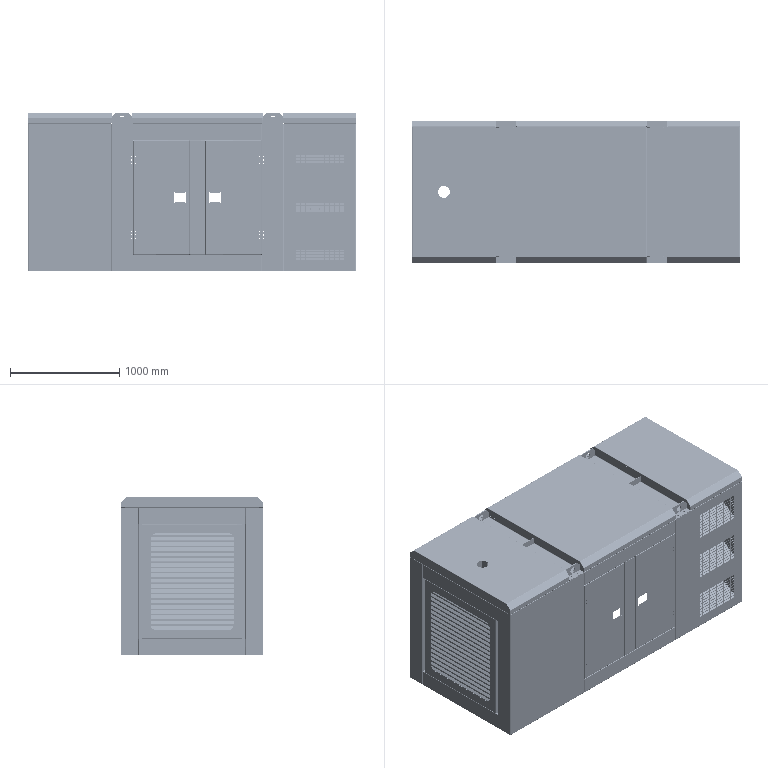Assembly | SolidWorks | mm | 126 component files | 130 solids | 11955 faces | box 3000 x 1300 x 1450 mm | volume 58582287 mm3 | plane 6546 | cylinder 5009 | spline 244 | cone 156 | commonest cylinder face diameters 6 x2539 10 x690 5 x576 8 x305 4 x293 9 x192 16 x116 7 x114
Bill of materials:
AirInletUpperBeam | 1 | Plain Carbon Steel | Rectangular panel with short bent flanges at the edges. A large grid of rectangular, rounded-corner slots sits in two equal side-by-side fields.
AirInletUpperBeamBaffle | 1 |  | Long prism-shaped shell with a vertical rear wall, two end walls and a sloped front face. The end profile is a right trapezoid.
AirInletVent | 1 | Plain Carbon Steel | Large rectangular panel with four fields of rectangular slots in a 2x2 layout. Narrow side flanges carry round holes.
AirInletVentBaffle | 2 |  | Long prism-shaped shell like unnamed part but with different proportions: rear wall, two end walls and a sloped front face.
Door | 4 | Plain Carbon Steel | Thin, flat rectangular plate with one rectangular cutout near one long edge and two groups of small oblong holes along the opposite long edge.
DoorStiffener | 8 | Plain Carbon Steel | Long straight channel with a C/U cross-section: a web and two parallel flanges with rounded bends.
BreakerDoor | 1 | Plain Carbon Steel | Thin, almost square flat plate. It has a central rounded-rectangle cutout, a rectangular cutout with slotted ends near one side, and four oblong slots along the opposite edge.
ElectricalCabinet | 1 | Plain Carbon Steel | Hat-section cover: a U-shaped box (face plus two side walls) with outward mounting flanges along both open edges. A horizontal obround slot runs through the face.
ElectricalCabinetBaffle | 1 | Plain Carbon Steel | Rectangular flat strip with a short bent lip at one end (L-profile). It has two round holes near the other end and one cylindrical boss or pin on the face.
CableClamp | 4 | Plain Carbon Steel | Thick U-shaped bracket or strap with a flat base, two parallel legs and radiused inner and outer bends.
ControlPanel | 1 | Plain Carbon Steel | Thin, flat rectangular plate with a large rectangular window, a narrow rectangular cutout with slotted ends, a row of three round holes, and four oblong slots along one edge.
ElectricalCabinetDoor | 1 | Plain Carbon Steel | Thin, flat rectangular plate with a large rounded-rectangle window near one end, a vertical obround slot, and four small slots along one long edge.
ElectricalCabinetDoorStiffener | 1 | Plain Carbon Steel | Long, straight C-channel profile of uniform thin wall. It has a flat web and two parallel flanges with rounded bends. No holes are visible.
ExhaustVent | 1 | Plain Carbon Steel | Square, thin frame-like plate with a large central opening shaped as a square with rounded corners. Narrow flanges or offset strips run along its edges, with small holes or slots spaced along two opposite edges.
Louver | 19 | Plain Carbon Steel | Long, narrow, thin strip bent along its length. In the end profile, a short straight leg joins a longer leg at an obtuse angle through a rounded bend.
FrontBeam | 2 | Plain Carbon Steel | Long, shallow, rectangular open tray or box section made of thin wall. A flat base has upturned walls on all four sides. Elongated slots are spaced along both long walls, and there are two slots in each end wall.
FrontSidePanel | 2 | Plain Carbon Steel | Large, flat, rectangular thin panel with a narrow return flange along one long edge and an L-shaped flange or lip along one end. Small holes run along the return flange, and slots are in the end flange.
FrontSidePanelReinforcementHorizontalRib | 2 |  | Long, straight L-angle profile of thin uniform wall. Two legs of about equal length meet at a rounded 90 degree bend. No holes are visible.
FrontSidePanelReinforcementVerticalRib | 2 |  | Long, slender L-angle profile with a rounded 90 degree bend. A single row of small holes runs along one leg.
hex nuts-style normal-grades ab gb | 12 |  | Hexagonal nut-like body with a central round through-bore. The hex corners are chamfered on both faces, which gives curved edges on the side faces.
FrontTopCover | 1 | Plain Carbon Steel | Large, rectangular thin cover plate with one round hole set off-center. A downturned flange with angled corner transitions runs along one edge, and a narrow flange with small holes and a return lip runs along an adjacent edge.
FrontTopCoverStiffener | 1 |  | Long, slender L-angle strip with a rounded 90 degree bend. Four elongated slots are evenly spaced along one leg.
HangingChannel | 2 | Plain Carbon Steel | Long U-channel or trough with a flat base, two tall parallel side walls and rounded bends. The ends of the side walls are cut at an angle. Small holes run along both side walls, and larger holes sit near each end of the base.
HangingChannelStiffener | 2 |  | Flat rectangular plate of uniform thickness. The two corners on one long edge are rounded, and the other two corners are square. No holes are visible.
LiftingLug | 4 | Plain Carbon Steel | Flat plate of constant thickness. Its outline has a straight bottom edge, two vertical sides and two angled (chamfered) upper corners. It has one large central round through-hole and a small rounded notch cut into the middle of the bottom edge.
HingeColumn | 4 | Plain Carbon Steel | Long, narrow formed sheet part. The end-on view shows a shallow U-shaped channel with a short outward-turned flange on one side. The base carries two obround slots at each end, and small hole groups appear along the side flange.
LiftingBasePlate | 8 | Plain Carbon Steel | Flat rectangular plate of uniform thickness with two obround through-slots, one near each end. Two corners are rounded and the opposite two are square.
LiftingVerticalBeam | 4 | Plain Carbon Steel | Long, straight, thin-walled U-channel with rounded inside and outside bends and a constant cross-section. No holes are visible.
LiftingVerticalBeamStiffener | 12 | Plain Carbon Steel | Plain flat rectangular plate of uniform thickness. Two corners on one long edge are rounded and there are no holes.
LongitudinalStiffeningChannelSteel | 2 | Plain Carbon Steel | Long, shallow, open-top tray or channel with low side walls and closed end walls. Each end wall has two obround slots.
MiddleBeam | 4 | Plain Carbon Steel | Long formed sheet beam. The end profile is a deep vertical web with a short return flange at the bottom and an offset upturned lip along the top. The top lip has a gap in the middle with two small slots, and the ends have bent tabs with two obround slots each.
MiddleColumn | 2 | Plain Carbon Steel | Long formed sheet profile shaped like a hat (top-hat). The section is a U-channel with outward flanges at both rims. The base has two obround slots at each end, and small holes are visible along one side.
MiddleTopCover | 1 | Plain Carbon Steel | Large, almost square flat panel with shallow formed edges on two opposite sides. The end view shows short angled bends that turn down into vertical lips, with a small return at one end. A row of small holes runs along one formed edge.
TopCoverStiffener | 2 | Plain Carbon Steel | Very long, slender C-shaped (lipless channel) profile with a rounded-corner rectangular section open on one side. No holes are visible.
RearLeftSidePlate | 1 | Plain Carbon Steel | L-shaped bent sheet panel. The large face has three rectangular grid arrays of small rectangular perforations, and the face meets a narrower side flange at a right-angle bend. Short edge returns and small holes or obround slots are present along the edges.
RearLeftSidePlateAirInletBaffle | 3 | Plain Carbon Steel | Thin sheet part with an open-box form: a back wall, two triangular or trapezoidal end walls, and a sloped base face. In the side view the profile tapers to a point. There are no holes or cutouts.
RearRightSidePanelVerticalRib1 | 1 | Plain Carbon Steel | Long, slender L-section angle strip that looks like bent sheet, with a rounded inside bend and three small holes evenly spaced along one leg.
RearRightSidePlate | 1 | Plain Carbon Steel | Flat rectangular panel that looks like bent sheet, with a large rectangular window cutout. It has one large round hole surrounded by four small holes near a top corner and a row of four round holes below the window. Its edges are folded into perimeter flanges, including a deeper flange down one long side, and the flanges carry small holes and oblong slots.
RearRightSidePlateDoorHorizontalRib | 2 | Plain Carbon Steel | Long narrow strip that looks like bent sheet: a flat top web with one long edge bent down into a flange. The web extends past the flange at both ends, forming end tabs or notches.
RearRightSidePlateDoorVerticalRib2 | 1 | Plain Carbon Steel | Long, slender L-section angle strip that looks like bent sheet, with a rounded inside bend and three small holes evenly spaced along one leg.
RearTopCover | 1 | Plain Carbon Steel | Shallow rectangular plate or cover with a flat top face and short side walls or flanges. The corners at both short ends are chamfered at an angle.
Mates:
1. coincident | FrontSidePlateAssembly-1/FrontSidePanel-1 face at (-416.713, -34.451, 675.478) dir (0, 0, -1) | FrontSidePlateAssembly-2/FrontSidePanel-1 face at (-416.713, 1223.549, 675.478) dir (0, 0, -1)
2. coincident | FrontSidePlateAssembly-1/FrontSidePanel-1 face at (-420.713, 123.549, 2025.478) dir (-1, 0, 0) | FrontSidePlateAssembly-2/FrontSidePanel-1 face at (-420.713, 1103.549, 675.478) dir (-1, 0, 0)
3. distance | FrontSidePlateAssembly-1/FrontSidePanel-1 face at (-420.713, -36.451, 2025.478) dir (0, -1, 0) | FrontSidePlateAssembly-2/FrontSidePanel-1 face at (-420.713, 1263.549, 675.478) dir (0, 1, 0)
4. coincident | FrontSidePlateAssembly-1/FrontSidePanel-1 face at (-420.713, -36.451, 2025.478) dir (0, -1, 0) | HingeColumn-1 face at (339.287, -36.451, 2025.478) dir (0, -1, 0)
5. coincident | FrontSidePlateAssembly-1/FrontSidePanel-1 face at (-416.713, -34.451, 675.478) dir (0, 0, -1) | HingeColumn-1 face at (343.287, -34.451, 675.478) dir (0, 0, -1)
6. coincident | FrontSidePlateAssembly-1/FrontSidePanel-1 face at (339.287, -36.451, 2025.478) dir (1, 0, 0) | HingeColumn-1 face at (339.287, 13.549, 2025.478) dir (-1, 0, 0)
7. coincident | HingeColumn-1 face at (343.287, -34.451, 675.478) dir (0, 0, -1) | MiddleBeam-1 face at (539.287, -36.451, 675.478) dir (0, 0, -1)
8. coincident | HingeColumn-1 face at (339.287, -36.451, 2025.478) dir (0, -1, 0) | MiddleBeam-1 face at (539.287, -36.451, 825.478) dir (0, -1, 0)
9. coincident | HingeColumn-1 face at (539.287, -36.451, 2025.478) dir (1, 0, 0) | MiddleBeam-1 face at (539.287, 3.549, 825.478) dir (-1, 0, 0)
10. coincident | MiddleBeam-1 face at (539.287, -36.451, 675.478) dir (0, 0, -1) | HingeColumn-2 face at (1915.287, 13.549, 675.478) dir (0, 0, -1)
11. coincident | MiddleBeam-1 face at (539.287, -36.451, 825.478) dir (0, -1, 0) | HingeColumn-2 face at (1919.287, -36.451, 675.478) dir (0, -1, 0)
12. coincident | MiddleBeam-1 face at (1719.287, 3.549, 825.478) dir (1, 0, 0) | HingeColumn-2 face at (1719.287, -36.451, 675.478) dir (-1, 0, 0)
13. coincident | HingeColumn-1 face at (539.287, -36.451, 2025.478) dir (1, 0, 0) | MiddleBeam-2 face at (539.287, 3.549, 1875.478) dir (-1, 0, 0)
14. coincident | HingeColumn-1 face at (339.287, -36.451, 2025.478) dir (0, -1, 0) | MiddleBeam-2 face at (1719.287, -36.451, 1875.478) dir (0, -1, 0)
15. coincident | HingeColumn-1 face at (343.287, 13.549, 2025.478) dir (0, 0, 1) | MiddleBeam-2 face at (1719.287, -36.451, 2025.478) dir (0, 0, 1)
16. coincident | MiddleBeam-1 face at (539.287, 3.549, 825.478) dir (0, 0, 1) | MiddleColumn-1 face at (1059.287, -34.451, 825.478) dir (0, 0, -1)
17. coincident | MiddleBeam-1 face at (539.287, -36.451, 825.478) dir (0, -1, 0) | MiddleColumn-1 face at (1059.287, -36.451, 1875.478) dir (0, -1, 0)
18. distance | HingeColumn-1 face at (539.287, -36.451, 2025.478) dir (1, 0, 0) | MiddleColumn-1 face at (1059.287, -34.451, 825.478) dir (-1, 0, 0)
19. coincident | HingeColumn-1 face at (339.287, -36.451, 2025.478) dir (0, -1, 0) | DoorAssembly-1/Door-1 face at (541.787, -36.451, 1872.978) dir (0, -1, 0)
20. distance | MiddleBeam-1 face at (539.287, 3.549, 825.478) dir (0, 0, 1) | DoorAssembly-1/Door-1 face at (541.787, -34.451, 827.978) dir (0, 0, -1)
21. distance | MiddleColumn-1 face at (1059.287, -34.451, 825.478) dir (-1, 0, 0) | DoorAssembly-1/Door-1 face at (1056.787, -34.451, 827.978) dir (1, 0, 0)
22. coincident | HingeColumn-2 face at (1919.287, -36.451, 675.478) dir (0, -1, 0) | DoorAssembly-2/Door-1 face at (1716.787, -36.451, 827.978) dir (0, -1, 0)
23. distance | HingeColumn-2 face at (1719.287, -36.451, 675.478) dir (-1, 0, 0) | DoorAssembly-2/Door-1 face at (1716.787, -34.451, 1872.978) dir (1, 0, 0)
24. distance | MiddleBeam-1 face at (539.287, 3.549, 825.478) dir (0, 0, 1) | DoorAssembly-2/Door-1 face at (1716.787, -34.451, 827.978) dir (0, 0, -1)
25. coincident | HingeColumn-2 face at (1915.287, 13.549, 677.478) dir (0, 0, 1) | LiftingVerticalBeamAssembly-1/LiftingBasePlate-2 face at (1753.287, -29.451, 677.478) dir (0, 0, -1)
26. coincident | HingeColumn-2 face at (1919.287, -34.451, 675.478) dir (0, 1, 0) | LiftingVerticalBeamAssembly-1/LiftingVerticalBeam-1 face at (1749.287, -34.451, 2022.478) dir (0, -1, 0)
27. distance | HingeColumn-2 face at (1919.287, 13.549, 675.478) dir (1, 0, 0) | LiftingVerticalBeamAssembly-1/LiftingVerticalBeam-1 face at (1889.287, -34.451, 2022.478) dir (1, 0, 0)
28. coincident | HingeColumn-1 face at (343.287, -34.451, 677.478) dir (0, 0, 1) | LiftingVerticalBeamAssembly-2/LiftingBasePlate-2 face at (373.287, -29.451, 677.478) dir (0, 0, -1)
29. coincident | HingeColumn-1 face at (339.287, -34.451, 2025.478) dir (0, 1, 0) | LiftingVerticalBeamAssembly-2/LiftingVerticalBeam-1 face at (369.287, -34.451, 2022.478) dir (0, -1, 0)
30. distance | HingeColumn-1 face at (339.287, 13.549, 2025.478) dir (-1, 0, 0) | LiftingVerticalBeamAssembly-2/LiftingVerticalBeam-1 face at (369.287, 19.549, 2022.478) dir (-1, 0, 0)
31. coincident | FrontSidePlateAssembly-1/FrontSidePanel-1 face at (-420.713, 123.549, 2025.478) dir (-1, 0, 0) | FrontBeam-1 face at (-420.713, 123.549, 675.478) dir (-1, 0, 0)
32. coincident | FrontSidePlateAssembly-1/FrontSidePanel-1 face at (-380.713, 123.549, 2025.478) dir (0, 1, 0) | FrontBeam-1 face at (-418.713, 123.549, 675.478) dir (0, -1, 0)
33. coincident | FrontSidePlateAssembly-2/FrontSidePanel-1 face at (-380.713, 1107.549, 675.478) dir (0, 0, -1) | FrontBeam-1 face at (-418.713, 123.549, 675.478) dir (0, 0, -1)
34. coincident | FrontSidePlateAssembly-1/FrontSidePanel-1 face at (-420.713, 123.549, 2025.478) dir (-1, 0, 0) | FrontBeam-2 face at (-420.713, 123.549, 1875.478) dir (-1, 0, 0)
35. coincident | FrontSidePlateAssembly-1/FrontSidePanel-1 face at (-380.713, 123.549, 2025.478) dir (0, 1, 0) | FrontBeam-2 face at (-418.713, 123.549, 1875.478) dir (0, -1, 0)
36. coincident | FrontSidePlateAssembly-1/FrontSidePanel-1 face at (-380.713, 119.549, 2025.478) dir (0, 0, 1) | FrontBeam-2 face at (-418.713, 123.549, 2025.478) dir (0, 0, 1)
37. coincident | FrontSidePlateAssembly-1/FrontSidePanel-1 face at (-420.713, 123.549, 2025.478) dir (-1, 0, 0) | ExhaustVentAssembly-1/ExhaustVent-1 face at (-420.713, 153.549, 1875.478) dir (-1, 0, 0)
38. coincident | FrontBeam-1 face at (-418.713, 123.549, 825.478) dir (0, 0, 1) | ExhaustVentAssembly-1/ExhaustVent-1 face at (-380.713, 153.549, 825.478) dir (0, 0, -1)
39. distance | FrontSidePlateAssembly-1/FrontSidePanel-1 face at (-380.713, 123.549, 2025.478) dir (0, 1, 0) | ExhaustVentAssembly-1/ExhaustVent-1 face at (-380.713, 153.549, 1875.478) dir (0, -1, 0)
40. coincident | MiddleColumn-3 face at (1199.287, 1263.549, 1875.478) dir (0, 1, 0) | DoorAssembly-4/Door-1 face at (541.787, 1263.549, 827.978) dir (0, 1, 0)
41. distance | HingeColumn-5 face at (539.287, 1263.549, 675.478) dir (1, 0, 0) | DoorAssembly-4/Door-1 face at (541.787, 1261.549, 1872.978) dir (-1, 0, 0)
42. distance | MiddleBeam-6 face at (1719.287, 1223.549, 825.478) dir (0, 0, 1) | DoorAssembly-4/Door-1 face at (541.787, 1261.549, 827.978) dir (0, 0, -1)
43. coincident | MiddleColumn-3 face at (1199.287, 1263.549, 1875.478) dir (0, 1, 0) | DoorAssembly-5/Door-1 face at (1716.787, 1263.549, 1872.978) dir (0, 1, 0)
44. distance | HingeColumn-6 face at (1719.287, 1263.549, 2025.478) dir (-1, 0, 0) | DoorAssembly-5/Door-1 face at (1716.787, 1261.549, 827.978) dir (1, 0, 0)
45. distance | MiddleBeam-5 face at (539.287, 1223.549, 1875.478) dir (0, 0, -1) | DoorAssembly-5/Door-1 face at (1716.787, 1261.549, 1872.978) dir (0, 0, 1)
46. coincident | HingeColumn-6 face at (1915.287, 1213.549, 2025.478) dir (0, 0, 1) | RearRightSidePlateAssembly-1/RearRightSidePlate-1 face at (1923.287, 1261.549, 2025.478) dir (0, 0, 1)
47. coincident | HingeColumn-6 face at (1919.287, 1263.549, 2025.478) dir (0, 1, 0) | RearRightSidePlateAssembly-1/RearRightSidePlate-1 face at (1919.287, 1263.549, 675.478) dir (0, 1, 0)
48. coincident | HingeColumn-6 face at (1919.287, 1213.549, 2025.478) dir (1, 0, 0) | RearRightSidePlateAssembly-1/RearRightSidePlate-1 face at (1919.287, 1263.549, 675.478) dir (-1, 0, 0)
49. coincident | HingeColumn-2 face at (1919.287, -36.451, 675.478) dir (0, -1, 0) | RearLeftSidePlateAssembly-2/RearLeftSidePlate-1 face at (1919.287, -36.451, 2025.478) dir (0, -1, 0)
50. coincident | HingeColumn-2 face at (1915.287, -34.451, 2025.478) dir (0, 0, 1) | RearLeftSidePlateAssembly-2/RearLeftSidePlate-1 face at (1923.287, 3.549, 2025.478) dir (0, 0, 1)
51. coincident | HingeColumn-2 face at (1919.287, 13.549, 675.478) dir (1, 0, 0) | RearLeftSidePlateAssembly-2/RearLeftSidePlate-1 face at (1919.287, -36.451, 2025.478) dir (-1, 0, 0)
52. coincident | RearLeftSidePlateAssembly-2/RearLeftSidePlate-1 face at (2539.287, -32.451, 2025.478) dir (0, 0, 1) | AirInletUpperBeamAssembly-1/AirInletUpperBeam-1 face at (2577.287, 1103.549, 2025.478) dir (0, 0, 1)
53. coincident | RearLeftSidePlateAssembly-2/RearLeftSidePlate-1 face at (2579.287, -36.451, 2025.478) dir (1, 0, 0) | AirInletUpperBeamAssembly-1/AirInletUpperBeam-1 face at (2579.287, 1103.549, 1625.478) dir (1, 0, 0)
54. coincident | RearRightSidePlateAssembly-1/RearRightSidePlate-1 face at (2579.287, 1103.549, 675.478) dir (0, -1, 0) | AirInletUpperBeamAssembly-1/AirInletUpperBeam-1 face at (2577.287, 1103.549, 1625.478) dir (0, 1, 0)
55. distance | RearRightSidePlateAssembly-1/RearRightSidePlate-1 face at (2539.287, 1259.549, 675.478) dir (0, 0, -1) | AirInletVentAssembly-1/AirInletVent-1 face at (2577.287, 154.549, 677.478) dir (0, 0, -1)
56. coincident | RearLeftSidePlateAssembly-2/RearLeftSidePlate-1 face at (2579.287, -36.451, 2025.478) dir (1, 0, 0) | AirInletVentAssembly-1/AirInletVent-1 face at (2579.287, 154.549, 677.478) dir (1, 0, 0)
57. distance | RearLeftSidePlateAssembly-2/RearLeftSidePlate-1 face at (2579.287, 123.549, 2025.478) dir (0, 1, 0) | AirInletVentAssembly-1/AirInletVent-1 face at (2544.287, 154.549, 677.478) dir (0, -1, 0)
58. coincident | RearRightSidePlateAssembly-1/RearRightSidePanelVerticalRib1-1 face at (1967.287, 1213.549, 677.978) dir (0, 1, 0) | ElectricalCabinetAssembly-1/CabinetAssembly-1/ElectricalCabinet-1 face at (2011.287, 1213.549, 1759.478) dir (0, -1, 0)
59. concentric | RearRightSidePlateAssembly-1/RearRightSidePlateDoorVerticalRib2-1 face at (2457.287, 1211.549, 1710.478) dir (0, 1, 0) r 5 | ElectricalCabinetAssembly-1/CabinetAssembly-1/ElectricalCabinet-1 face at (2457.287, 1205.549, 1710.478) dir (0, 1, 0) r 5
60. concentric | RearRightSidePlateAssembly-1/RearRightSidePanelVerticalRib1-1 face at (1981.287, 1211.549, 1710.478) dir (0, 1, 0) r 5 | ElectricalCabinetAssembly-1/CabinetAssembly-1/ElectricalCabinet-1 face at (1981.287, 1205.549, 1710.478) dir (0, 1, 0) r 5
61. coincident | RearRightSidePlateAssembly-1/RearRightSidePlate-1 face at (1919.287, 1263.549, 675.478) dir (0, 1, 0) | ElectricalCabinetDoorAssembly-1/ElectricalCabinetDoor-1 face at (1971.787, 1263.549, 927.978) dir (0, 1, 0)
62. distance | RearRightSidePlateAssembly-1/RearRightSidePlateDoorHorizontalRib-1 face at (1991.287, 1261.549, 1775.478) dir (0, 0, -1) | ElectricalCabinetDoorAssembly-1/ElectricalCabinetDoor-1 face at (1971.787, 1261.549, 1772.978) dir (0, 0, 1)
63. distance | RearRightSidePlateAssembly-1/RearRightSidePanelVerticalRib1-1 face at (1969.287, 1261.549, 677.978) dir (1, 0, 0) | ElectricalCabinetDoorAssembly-1/ElectricalCabinetDoor-1 face at (1971.787, 1261.549, 1772.978) dir (-1, 0, 0)
64. coincident | HingeColumn-5 face at (343.287, 1261.549, 2025.478) dir (0, 0, 1) | HangingChannelAssembly-2/HangingChannel-1 face at (539.287, 1263.549, 2025.478) dir (0, 0, -1)
65. coincident | HingeColumn-5 face at (339.287, 1263.549, 675.478) dir (0, 1, 0) | HangingChannelAssembly-2/HangingChannel-1 face at (539.287, 1263.549, 2029.478) dir (0, 1, 0)
66. coincident | HingeColumn-5 face at (339.287, 1213.549, 675.478) dir (-1, 0, 0) | HangingChannelAssembly-2/HangingChannel-1 face at (339.287, -36.451, 2029.478) dir (-1, 0, 0)
67. coincident | HingeColumn-6 face at (1915.287, 1213.549, 2025.478) dir (0, 0, 1) | HangingChannelAssembly-3/HangingChannel-1 face at (1719.287, -36.451, 2025.478) dir (0, 0, -1)
68. coincident | HingeColumn-6 face at (1919.287, 1263.549, 2025.478) dir (0, 1, 0) | HangingChannelAssembly-3/HangingChannel-1 face at (1719.287, 1263.549, 2029.478) dir (0, 1, 0)
69. coincident | HingeColumn-6 face at (1919.287, 1213.549, 2025.478) dir (1, 0, 0) | HangingChannelAssembly-3/HangingChannel-1 face at (1919.287, 1263.549, 2029.478) dir (1, 0, 0)
70. coincident | HangingChannelAssembly-3/HangingChannel-1 face at (1719.287, -36.451, 2025.478) dir (0, 0, -1) | LongitudinalStiffeningChannelSteel-1 face at (1719.287, 1191.549, 2025.478) dir (0, 0, -1)
71. coincident | HangingChannelAssembly-2/HangingChannel-1 face at (539.287, -36.451, 2122.478) dir (1, 0, 0) | LongitudinalStiffeningChannelSteel-1 face at (539.287, 1120.549, 2035.478) dir (-1, 0, 0)
72. distance | MiddleBeam-5 face at (539.287, 1263.549, 1875.478) dir (0, 1, 0) | LongitudinalStiffeningChannelSteel-1 face at (1719.287, 1191.549, 2025.478) dir (0, 1, 0)
73. coincident | FrontBeam-2 face at (-418.713, 123.549, 2025.478) dir (0, 0, 1) | FrontTopCoverAssembly-1/FrontTopCover-1 face at (339.287, 1263.549, 2025.478) dir (0, 0, -1)
74. coincident | FrontBeam-2 face at (-420.713, 123.549, 1875.478) dir (-1, 0, 0) | FrontTopCoverAssembly-1/FrontTopCover-1 face at (-420.713, 1211.892, 2123.478) dir (-1, 0, 0)
75. coincident | FrontSidePlateAssembly-1/FrontSidePanel-1 face at (-420.713, -36.451, 2025.478) dir (0, -1, 0) | FrontTopCoverAssembly-1/FrontTopCover-1 face at (-420.713, -36.451, 2025.478) dir (0, -1, 0)
76. coincident | MiddleBeam-2 face at (1719.287, -36.451, 2025.478) dir (0, 0, 1) | MiddleTopCoverAssembly-1/MiddleTopCover-1 face at (1719.287, 3.549, 2025.478) dir (0, 0, -1)
77. coincident | MiddleBeam-2 face at (1719.287, -36.451, 1875.478) dir (0, -1, 0) | MiddleTopCoverAssembly-1/MiddleTopCover-1 face at (1719.287, -36.451, 2025.478) dir (0, -1, 0)
78. distance | HangingChannelAssembly-3/HangingChannel-1 face at (1723.287, 1263.549, 2122.478) dir (1, 0, 0) | MiddleTopCoverAssembly-1/MiddleTopCover-1 face at (1724.287, 15.206, 2123.478) dir (-1, 0, 0)
79. coincident | RearLeftSidePlateAssembly-2/RearLeftSidePlate-1 face at (1923.287, 3.549, 2025.478) dir (0, 0, 1) | RearTopCoverAssembly-1/RearTopCover-1 face at (2579.287, 3.549, 2025.478) dir (0, 0, -1)
80. coincident | AirInletUpperBeamAssembly-1/AirInletUpperBeam-1 face at (2579.287, 1103.549, 1625.478) dir (1, 0, 0) | RearTopCoverAssembly-1/RearTopCover-1 face at (2579.287, 15.206, 2123.478) dir (1, 0, 0)
81. coincident | RearLeftSidePlateAssembly-2/RearLeftSidePlate-1 face at (1919.287, -36.451, 2025.478) dir (0, -1, 0) | RearTopCoverAssembly-1/RearTopCover-1 face at (2579.287, -36.451, 2025.478) dir (0, -1, 0)
82. coincident | AirInletUpperBeam-1 face at (-738.997, 97.614, 1368.825) dir (0, 1, 0) | AirInletUpperBeamBaffle-2 face at (185.003, 97.614, 1023.825) dir (0, -1, 0)
83. distance | AirInletUpperBeam-1 face at (-656.997, 97.614, 1272.325) dir (1, 0, 0) | AirInletUpperBeamBaffle-2 face at (-682.997, 247.614, 1227.222) dir (1, 0, 0)
84. distance | AirInletUpperBeam-1 face at (-384.497, 97.614, 1078.825) dir (0, 0, 1) | AirInletUpperBeamBaffle-2 face at (185.003, 249.614, 1023.825) dir (0, 0, -1)
85. coincident | AirInletVent-1 face at (-651.143, 76.053, 1533) dir (0, 1, 0) | AirInletVentBaffle-4 face at (-537.707, 76.053, 640) dir (0, -1, 0)
86. distance | AirInletVentBaffle-4 face at (-538.861, 196.053, 640) dir (0, 0, -1) | AirInletVent-1 face at (74.857, 76.053, 666) dir (0, 0, 1)
87. distance | AirInletVent-1 face at (-318.143, 76.053, 939) dir (-1, 0, 0) | AirInletVentBaffle-4 face at (-268.143, 198.053, 1510) dir (1, 0, 0)
88. parallel | Door-1 face at (207.586, 100.107, 573.135) dir (1, 0, 0) | DoorStiffener-1 face at (-297.414, 118.107, 1294.135) dir (-1, 0, 0)
89. distance | DoorStiffener-1 face at (-297.414, 118.107, 1294.135) dir (-1, 0, 0) | Door-1 face at (-307.414, 100.107, 573.135) dir (-1, 0, 0)
90. coincident | Door-1 face at (-307.414, 100.107, 1618.135) dir (0, 1, 0) | DoorStiffener-1 face at (-297.414, 100.107, 1298.135) dir (0, -1, 0)
91. distance | DoorStiffener-1 face at (-297.414, 120.107, 1298.135) dir (0, 0, 1) | Door-1 face at (-307.414, 100.107, 1618.135) dir (0, 0, 1)
92. coincident | Door-1 face at (-307.414, 100.107, 1618.135) dir (0, 1, 0) | DoorStiffener-2 face at (-302.414, 100.107, 933.135) dir (0, -1, 0)
93. distance | DoorStiffener-2 edge at (197.586, 116.107, 933.135) dir (0, -1, 0) | Door-1 face at (207.586, 100.107, 573.135) dir (1, 0, 0)
94. distance | Door-1 face at (-307.414, 100.107, 573.135) dir (0, 0, -1) | DoorStiffener-2 face at (-302.414, 100.107, 893.135) dir (0, 0, -1)
95. coincident | CabinetAssembly-1/ElectricalCabinet-1 face at (-270.686, -48.594, 510) dir (0, -1, 0) | ControlPanelAssembly-1/ControlPanel-1 face at (-268.186, -48.594, 1328) dir (0, 1, 0)
96. coincident | CabinetAssembly-1/ElectricalCabinet-1 face at (-270.686, -60.594, 1328) dir (0, 0, 1) | ControlPanelAssembly-1/ControlPanel-1 face at (143.814, -60.594, 1328) dir (0, 0, 1)
97. distance | CabinetAssembly-1/ElectricalCabinet-1 face at (-270.686, -60.594, 1328) dir (1, 0, 0) | ControlPanelAssembly-1/ControlPanel-1 face at (-268.186, -60.594, 1328) dir (-1, 0, 0)
98. coincident | CabinetAssembly-1/ElectricalCabinetBaffle-1 face at (-269.686, -48.594, 971) dir (0, -1, 0) | BreakerDoor-2 face at (143.814, -48.594, 512.5) dir (0, 1, 0)
99. distance | BreakerDoor-2 face at (143.814, -60.594, 965.5) dir (0, 0, 1) | ControlPanelAssembly-1/ControlPanel-1 face at (143.814, -60.594, 968) dir (0, 0, -1)
100. distance | CabinetAssembly-1/ElectricalCabinet-1 face at (-270.686, -60.594, 1328) dir (1, 0, 0) | BreakerDoor-2 face at (-268.186, -60.594, 965.5) dir (-1, 0, 0)
101. coincident | ElectricalCabinet-1 face at (-321.77, 87.808, 1338) dir (0, -1, 0) | ElectricalCabinetBaffle-1 face at (-318.77, 87.808, 983) dir (0, 1, 0)
102. coincident | ElectricalCabinet-1 face at (94.23, 87.808, 1338) dir (-1, 0, 0) | ElectricalCabinetBaffle-1 face at (94.23, 85.808, 983) dir (1, 0, 0)
103. distance | ElectricalCabinetBaffle-1 face at (-318.77, 85.808, 983) dir (0, 0, 1) | ElectricalCabinet-1 face at (-321.77, -52.192, 1338) dir (0, 0, 1)
104. coincident | ControlPanel-1 face at (-322.995, -149.043, 466.32) dir (0, 0, -1) | CableClamp-1 face at (-129.995, -109.043, 466.32) dir (0, 0, 1)
105. distance | ControlPanel-1 face at (-23.995, -79.043, 466.32) dir (0, 1, 0) | CableClamp-1 face at (-105.995, -109.043, 460.32) dir (0, 1, 0)
106. distance | CableClamp-1 face at (-131.995, -109.043, 466.32) dir (-1, 0, 0) | ControlPanel-1 face at (-322.995, -149.043, 468.32) dir (-1, 0, 0)
107. coincident | ControlPanel-1 face at (-322.995, -149.043, 466.32) dir (0, 0, -1) | CableClamp-2 face at (-244.995, -22.043, 466.32) dir (0, 0, 1)
108. distance | CableClamp-2 face at (-244.995, 1.957, 460.32) dir (-1, 0, 0) | ControlPanel-1 face at (-209.995, -79.043, 466.32) dir (1, 0, 0)
109. distance | ControlPanel-1 face at (-23.995, -79.043, 466.32) dir (0, 1, 0) | CableClamp-2 face at (-244.995, -24.043, 466.32) dir (0, -1, 0)
110. coincident | ElectricalCabinetDoor-1 face at (-422.942, 43.551, 1368.135) dir (0, 1, 0) | ElectricalCabinetDoorStiffener-1 face at (67.058, 43.551, 921.135) dir (0, -1, 0)
111. distance | ElectricalCabinetDoorStiffener-1 face at (-412.942, 61.551, 919.135) dir (-1, 0, 0) | ElectricalCabinetDoor-1 face at (-422.942, 43.551, 523.135) dir (-1, 0, 0)
112. distance | ElectricalCabinetDoor-1 face at (-422.942, 43.551, 523.135) dir (0, 0, -1) | ElectricalCabinetDoorStiffener-1 face at (67.058, 63.551, 883.135) dir (0, 0, -1)
113. coincident | ExhaustVent-1 face at (-628.17, 92.803, 1536) dir (0, 1, 0) | Louver-1 face at (351.83, 92.803, 1533) dir (0, -1, 0)
114. distance | Louver-1 face at (351.83, 94.803, 1533) dir (1, 0, 0) | ExhaustVent-1 face at (421.83, 130.803, 1536) dir (1, 0, 0)
115. distance | Louver-1 face at (338.487, 96.803, 619) dir (0, 0, -1) | ExhaustVent-1 face at (421.83, 92.803, 618) dir (0, 0, 1)
116. coincident | FrontSidePanel-1 face at (-740.849, 8.457, 2125.478) dir (0, 1, 0) | FrontSidePanelReinforcementVerticalRib-1 face at (-538.849, 8.457, 2122.978) dir (0, -1, 0)
117. distance | FrontSidePanel-1 face at (-740.849, 166.457, 2125.478) dir (-1, 0, 0) | FrontSidePanelReinforcementVerticalRib-1 face at (-540.849, 48.457, 2122.978) dir (-1, 0, 0)
118. distance | FrontSidePanelReinforcementVerticalRib-1 face at (-542.849, 12.457, 2122.978) dir (0, 0, 1) | FrontSidePanel-1 face at (-736.849, 46.457, 2123.478) dir (0, 0, -1)
119. coincident | FrontSidePanel-1 face at (-740.849, 8.457, 2125.478) dir (0, 1, 0) | FrontSidePanelReinforcementHorizontalRib-1 face at (-538.849, 8.457, 1425.478) dir (0, -1, 0)
120. coincident | FrontSidePanelReinforcementVerticalRib-1 face at (-538.849, 48.457, 2122.978) dir (1, 0, 0) | FrontSidePanelReinforcementHorizontalRib-1 face at (-538.849, 12.457, 1423.478) dir (-1, 0, 0)
121. distance | FrontSidePanelReinforcementHorizontalRib-1 face at (-538.849, 8.457, 1425.478) dir (0, 0, 1) | FrontSidePanel-1 face at (-736.849, 46.457, 2125.478) dir (0, 0, 1)
122. coincident | FrontSidePanel-1 face at (-698.849, 194.457, 2125.478) dir (1, 0, 0) | hex nuts-style normal-grades ab gb-1 face at (-698.849, 153.957, 959.601) dir (-1, 0, 0)
123. concentric | FrontSidePanel-1 face at (-698.849, 181.457, 975.478) dir (-1, 0, 0) r 4.5 | hex nuts-style normal-grades ab gb-1 face at (-698.849, 181.457, 975.478) dir (1, 0, 0) r 17.5
124. coincident | FrontTopCover-1 face at (-723.209, 181.253, 1683.5) dir (0, -1, 0) | FrontTopCoverStiffener-1 face at (-723.209, 181.253, 1483.5) dir (0, 1, 0)
125. distance | FrontTopCover-1 face at (-721.552, 181.253, 1683.5) dir (0, 0, 1) | FrontTopCoverStiffener-1 face at (-723.209, 181.253, 1483.5) dir (0, 0, 1)
126. distance | FrontTopCover-1 face at (-773.209, 83.253, 1683.5) dir (-1, 0, 0) | FrontTopCoverStiffener-1 face at (-723.209, 179.253, 1479.5) dir (-1, 0, 0)
127. coincident | HangingChannel-1 face at (-338.973, 553, 1544.5) dir (0, 0, -1) | LiftingLug-2 face at (-334.973, -683, 1544.5) dir (0, 0, 1)
128. coincident | HangingChannel-1 face at (-142.973, -747, 1544.5) dir (-1, 0, 0) | LiftingLug-2 face at (-142.973, -683, 1544.5) dir (1, 0, 0)
129. distance | LiftingLug-2 face at (-334.973, -693, 1544.5) dir (0, -1, 0) | HangingChannel-1 face at (-142.973, -743, 1544.5) dir (0, -1, 0)
130. coincident | HangingChannel-1 face at (-338.973, 553, 1544.5) dir (0, 0, -1) | HangingChannelStiffener-1 face at (-324.973, -94.5, 1544.5) dir (0, 0, 1)
131. coincident | HangingChannel-1 face at (-334.973, -747, 1451.5) dir (1, 0, 0) | HangingChannelStiffener-1 face at (-334.973, -94.5, 1534.5) dir (-1, 0, 0)
132. distance | HangingChannelStiffener-1 face at (-324.973, -99.5, 1534.5) dir (0, -1, 0) | HangingChannel-1 face at (-338.973, -747, 1544.5) dir (0, -1, 0)
133. coincident | LiftingVerticalBeam-1 face at (-75.046, -16.757, 745) dir (0, 0, 1) | LiftingBasePlate-1 face at (-80.046, -15.757, 745) dir (0, 0, 1)
134. coincident | LiftingVerticalBeam-1 face at (51.954, 33.243, 745) dir (0, 1, 0) | LiftingBasePlate-1 face at (-80.046, 33.243, 740) dir (0, 1, 0)
135. coincident | LiftingVerticalBeam-1 face at (51.954, -20.757, 745) dir (-1, 0, 0) | LiftingBasePlate-1 face at (51.954, 33.243, 740) dir (1, 0, 0)
136. coincident | LiftingVerticalBeam-1 face at (46.954, -16.757, -600) dir (0, 0, -1) | LiftingBasePlate-2 face at (-80.046, -15.757, -600) dir (0, 0, -1)
137. coincident | LiftingVerticalBeam-1 face at (51.954, 33.243, 745) dir (0, 1, 0) | LiftingBasePlate-2 face at (-80.046, 33.243, -600) dir (0, 1, 0)
138. coincident | LiftingVerticalBeam-1 face at (-80.046, 33.243, 745) dir (1, 0, 0) | LiftingBasePlate-2 face at (-80.046, 33.243, -600) dir (-1, 0, 0)
139. distance | LiftingVerticalBeamStiffener-1 face at (-80.046, -16.757, -265) dir (0, 0, -1) | LiftingBasePlate-2 face at (-80.046, -15.757, -600) dir (0, 0, -1)
140. coincident | LiftingVerticalBeam-1 face at (-80.046, 33.243, 745) dir (1, 0, 0) | LiftingVerticalBeamStiffener-1 face at (-80.046, 32.243, -265) dir (-1, 0, 0)
141. coincident | LiftingVerticalBeam-1 face at (-84.046, -16.757, 745) dir (0, 1, 0) | LiftingVerticalBeamStiffener-1 face at (-80.046, -16.757, -265) dir (0, -1, 0)
142. coincident | MiddleTopCover-1 face at (-833.983, 147.305, 2022) dir (0, -1, 0) | TopCoverStiffener-1 face at (366.017, 147.305, 1447) dir (0, 1, 0)
143. distance | MiddleTopCover-1 face at (416.017, 49.305, 2022) dir (1, 0, 0) | TopCoverStiffener-1 face at (366.017, 145.305, 1433) dir (1, 0, 0)
144. distance | MiddleTopCover-1 face at (-832.326, 147.305, 2029) dir (0, 0, 1) | TopCoverStiffener-1 face at (366.017, 147.305, 1429) dir (0, 0, -1)
145. coincident | RearLeftSidePlate-1 face at (-340.706, -40.716, 2125.166) dir (0, 1, 0) | RearLeftSidePlateAirInletBaffle-1 face at (-272.706, -40.716, 1185.166) dir (0, -1, 0)
146. distance | RearLeftSidePlateAirInletBaffle-1 face at (247.294, 140.284, 969.089) dir (1, 0, 0) | RearLeftSidePlate-1 face at (319.294, -42.716, 2125.166) dir (1, 0, 0)
147. distance | RearLeftSidePlateAirInletBaffle-1 face at (-272.706, 140.284, 1185.166) dir (0, 0, 1) | RearLeftSidePlate-1 face at (-336.706, -40.716, 775.166) dir (0, 0, -1)
148. coincident | RearLeftSidePlate-1 face at (282.294, 117.284, 2125.166) dir (-1, 0, 0) | hex nuts-style normal-grades ab gb-1 face at (282.294, 104.784, 841.043) dir (1, 0, 0)
149. concentric | RearLeftSidePlate-1 face at (282.294, 132.284, 825.166) dir (1, 0, 0) r 4.5 | hex nuts-style normal-grades ab gb-1 face at (282.294, 132.284, 825.166) dir (-1, 0, 0) r 17.5
150. coincident | RearRightSidePlate-1 face at (-322.635, -113.837, 2125.166) dir (0, 1, 0) | RearRightSidePanelVerticalRib1-1 face at (-272.635, -113.837, 2122.666) dir (0, -1, 0)
151. distance | RearRightSidePanelVerticalRib1-1 face at (-270.635, -65.837, 777.666) dir (0, 0, -1) | RearRightSidePlate-1 face at (-318.635, -113.837, 777.166) dir (0, 0, 1)
152. coincident | RearRightSidePlate-1 face at (-272.635, -113.837, 1025.166) dir (1, 0, 0) | RearRightSidePanelVerticalRib1-1 face at (-272.635, -113.837, 2122.666) dir (1, 0, 0)
153. coincident | RearRightSidePlate-1 face at (-322.635, -113.837, 2125.166) dir (0, 1, 0) | RearRightSidePlateDoorVerticalRib2-1 face at (227.365, -113.837, 777.666) dir (0, -1, 0)
154. coincident | RearRightSidePlate-1 face at (227.365, -113.837, 1025.166) dir (-1, 0, 0) | RearRightSidePlateDoorVerticalRib2-1 face at (227.365, -113.837, 777.666) dir (-1, 0, 0)
155. distance | RearRightSidePlate-1 face at (-318.635, -113.837, 777.166) dir (0, 0, 1) | RearRightSidePlateDoorVerticalRib2-1 face at (225.365, -67.837, 777.666) dir (0, 0, -1)
156. coincident | RearRightSidePlate-1 face at (-322.635, -113.837, 2125.166) dir (0, 1, 0) | RearRightSidePlateDoorHorizontalRib-1 face at (-250.635, -113.837, 1025.166) dir (0, -1, 0)
157. coincident | RearRightSidePlate-1 face at (227.365, -113.837, 1025.166) dir (0, 0, 1) | RearRightSidePlateDoorHorizontalRib-1 face at (-250.635, -113.837, 1025.166) dir (0, 0, 1)
158. coincident | RearRightSidePanelVerticalRib1-1 face at (-250.635, -63.837, 2122.666) dir (1, 0, 0) | RearRightSidePlateDoorHorizontalRib-1 face at (-250.635, -67.837, 1025.166) dir (-1, 0, 0)
159. coincident | RearRightSidePlate-1 face at (-322.635, -113.837, 2125.166) dir (0, 1, 0) | RearRightSidePlateDoorHorizontalRib-2 face at (205.365, -113.837, 1875.166) dir (0, -1, 0)
160. coincident | RearRightSidePlate-1 face at (227.365, -113.837, 1875.166) dir (0, 0, -1) | RearRightSidePlateDoorHorizontalRib-2 face at (205.365, -113.837, 1875.166) dir (0, 0, -1)
161. coincident | RearRightSidePlateDoorVerticalRib2-1 face at (205.365, -63.837, 777.666) dir (-1, 0, 0) | RearRightSidePlateDoorHorizontalRib-2 face at (205.365, -67.837, 1875.166) dir (1, 0, 0)
162. coincident | RearRightSidePlate-1 face at (300.365, 44.163, 2125.166) dir (-1, 0, 0) | hex nuts-style normal-grades ab gb-1 face at (300.365, 31.663, 1241.043) dir (1, 0, 0)
163. concentric | RearRightSidePlate-1 face at (300.365, 59.163, 1225.166) dir (1, 0, 0) r 4.5 | hex nuts-style normal-grades ab gb-1 edge at (294.978, 59.163, 1225.166) dir (1, 0, 0) r 3.458
164. coincident | RearTopCover-1 face at (-897.034, 191.441, 1763.5) dir (0, -1, 0) | TopCoverStiffener-1 face at (302.966, 191.441, 1433.5) dir (0, 1, 0)
165. distance | TopCoverStiffener-1 face at (-897.034, 189.441, 1429.5) dir (-1, 0, 0) | RearTopCover-1 face at (-947.034, 93.441, 1763.5) dir (-1, 0, 0)
166. distance | RearTopCover-1 face at (-895.377, 191.441, 1763.5) dir (0, 0, 1) | TopCoverStiffener-1 edge at (302.966, 165.441, 1433.5) dir (-1, 0, 0)